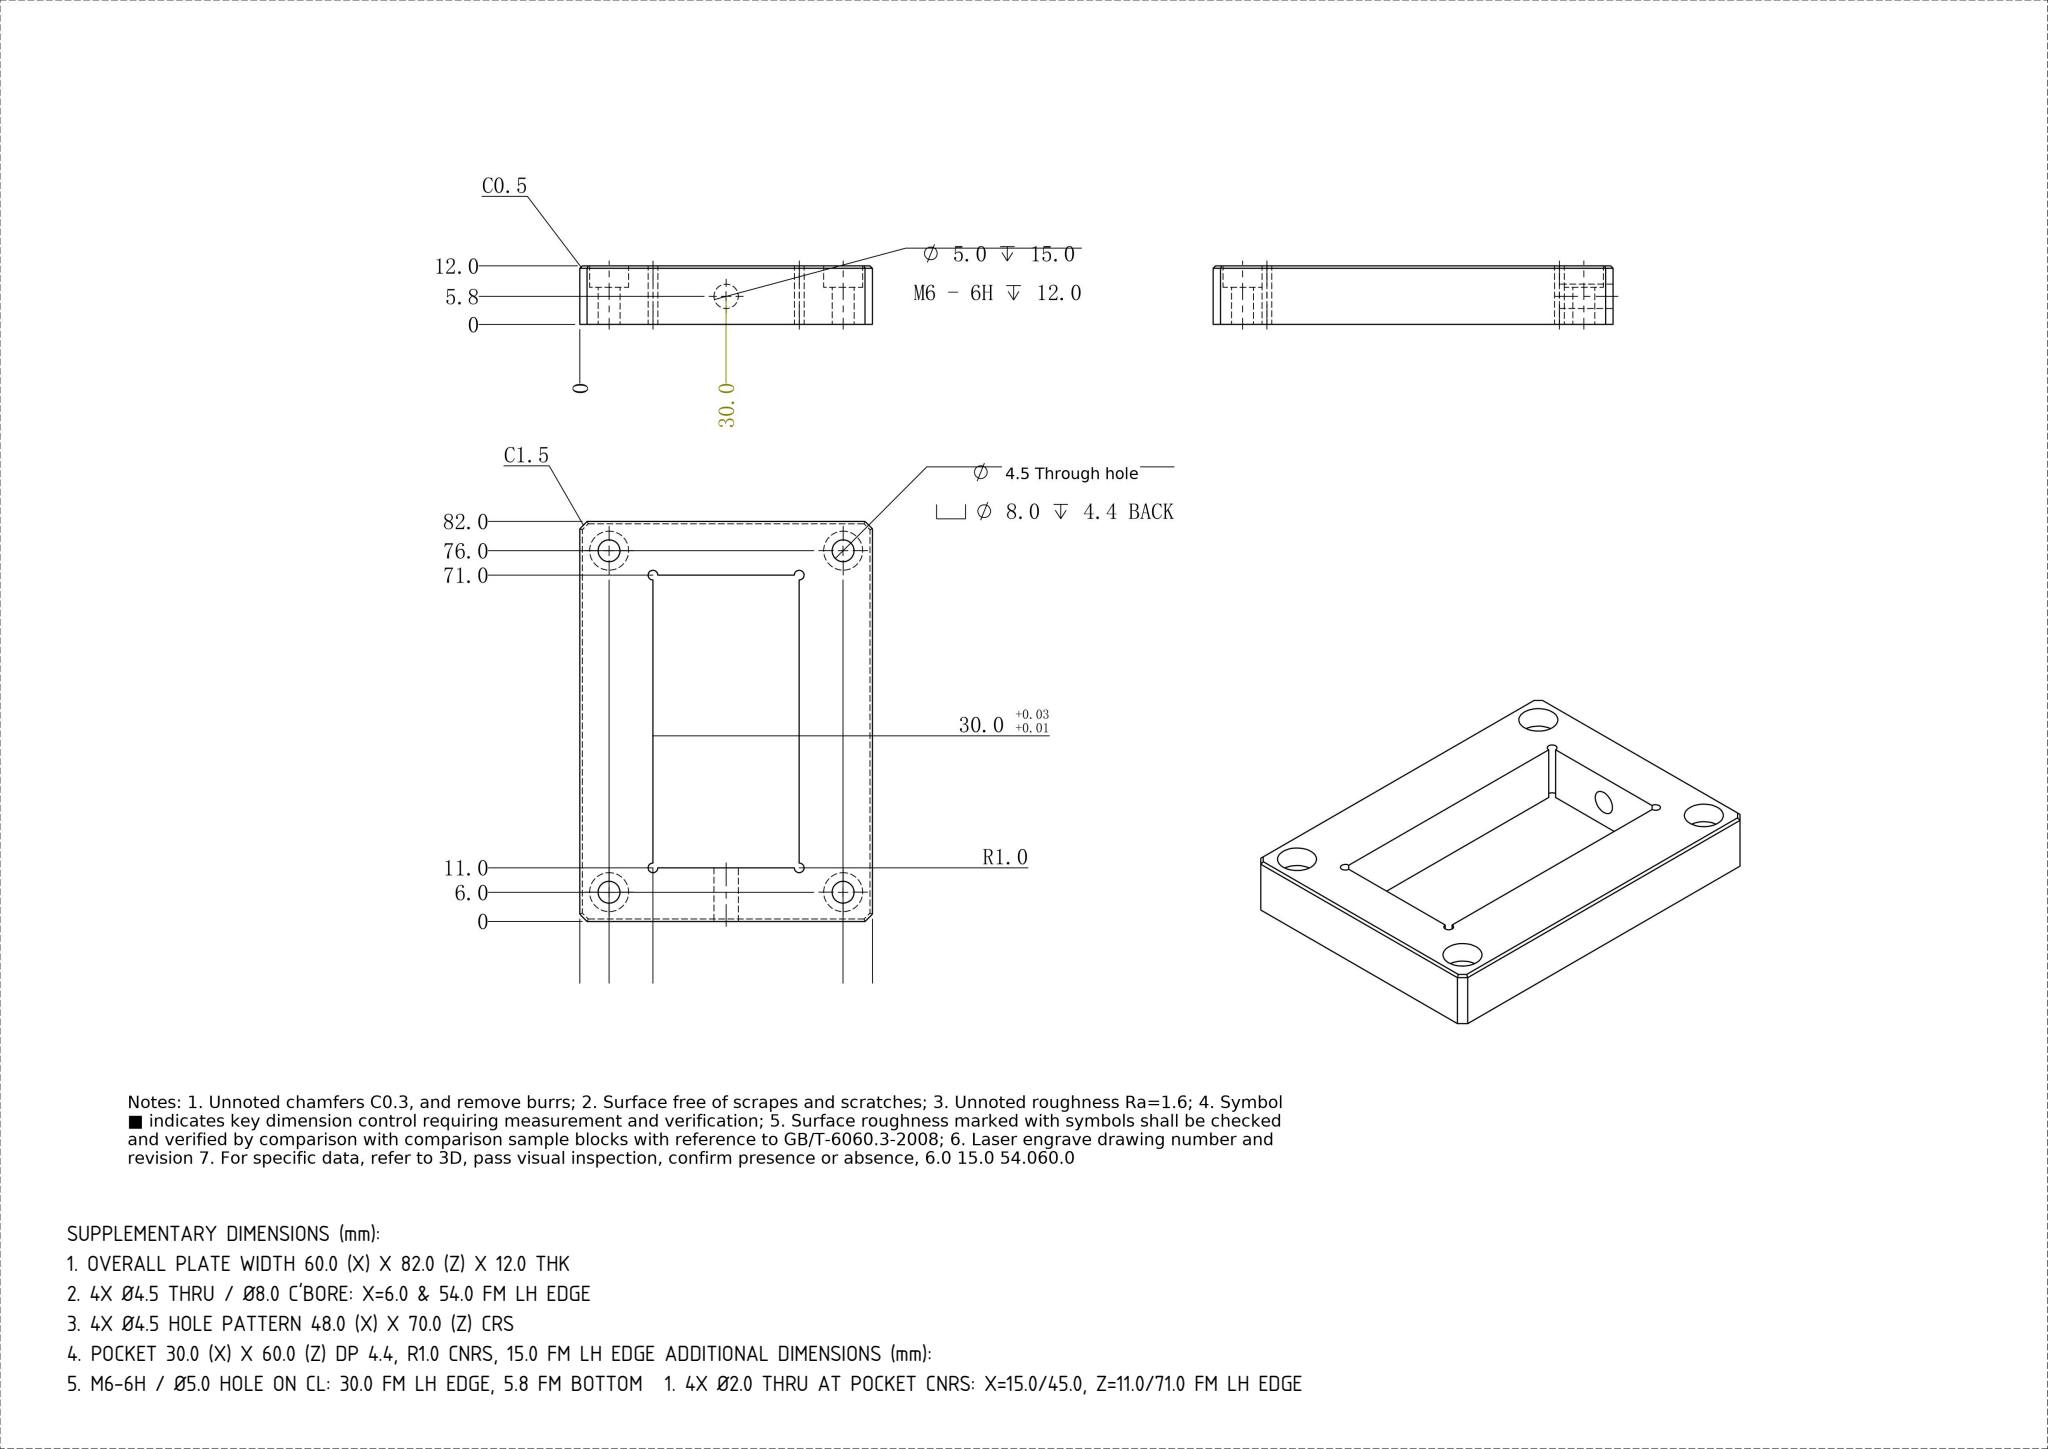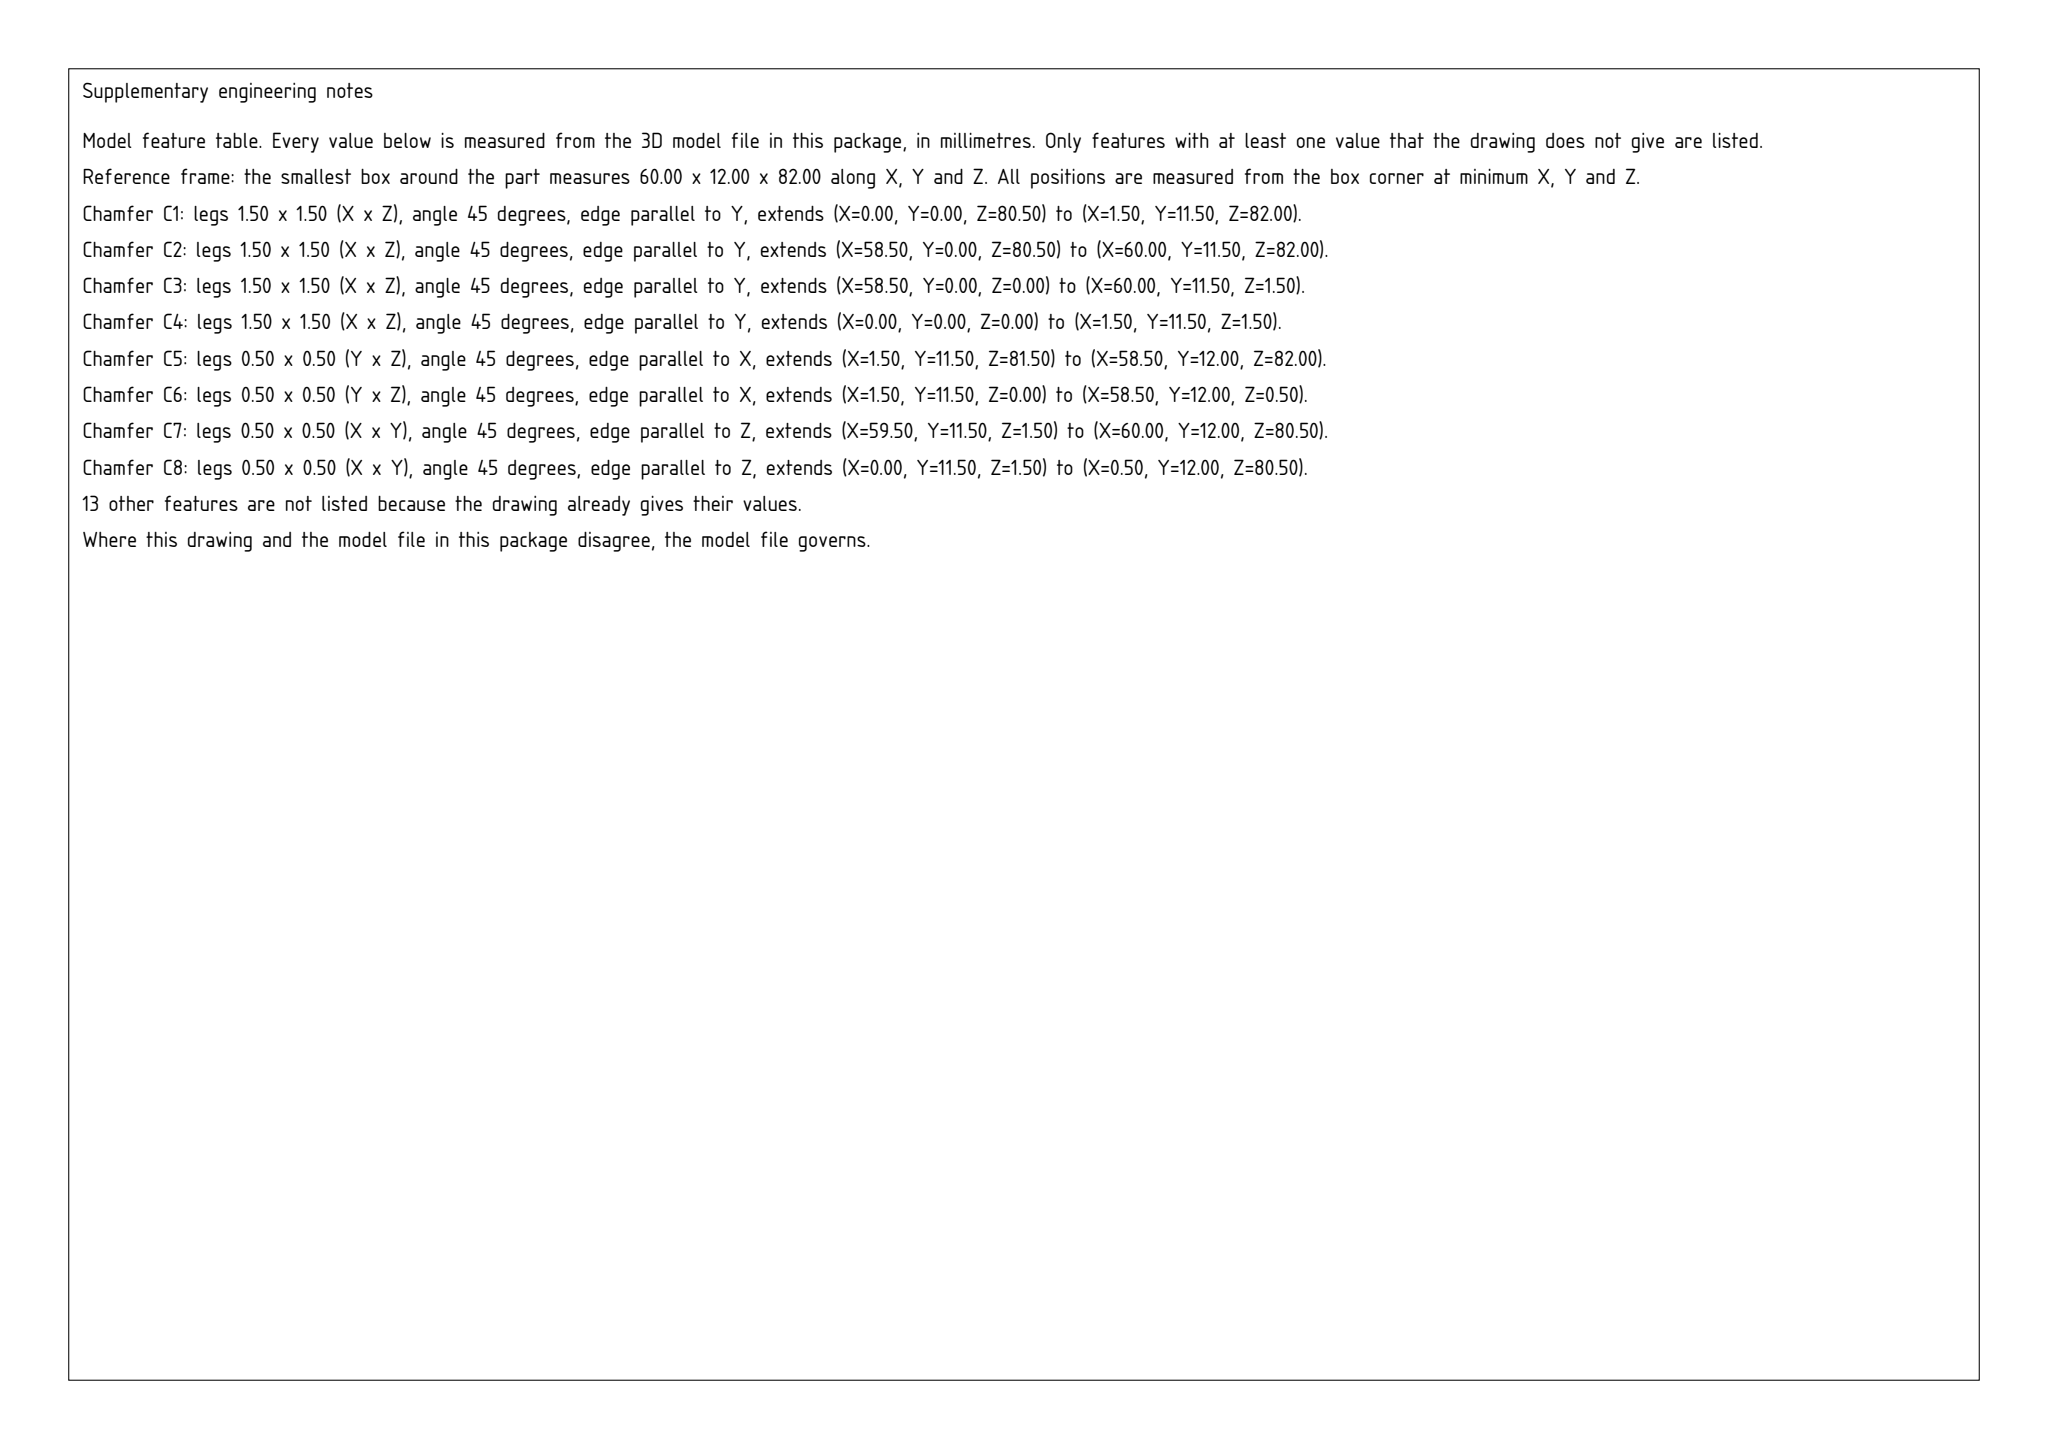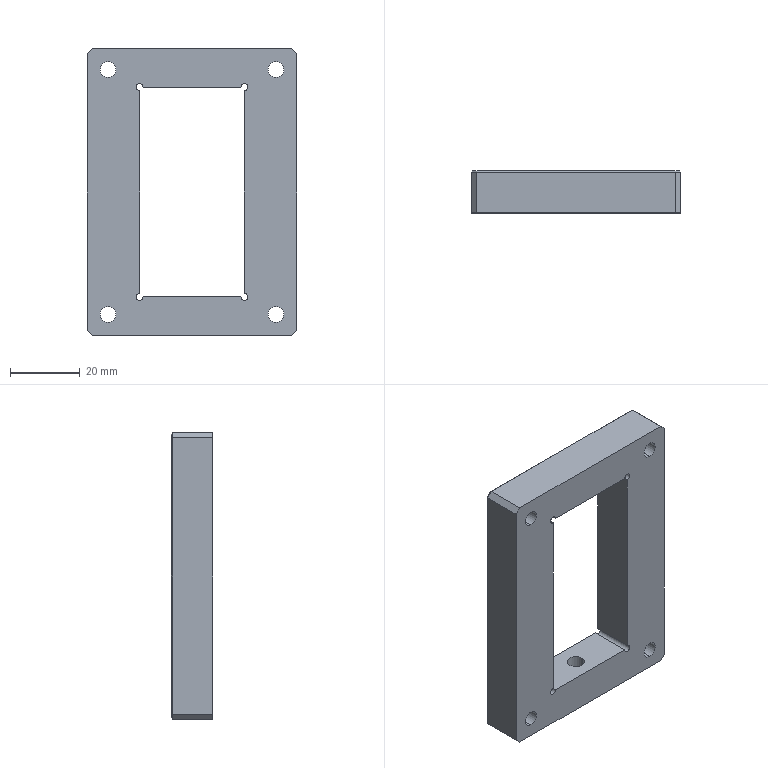Part | SolidWorks | mm | 1 solid | 50 faces | box 60 x 12 x 82 mm | volume 35654 mm3 | plane 26 | cylinder 24 | commonest cylinder face diameters 8 x8 4.5 x8 2 x6 5 x2
build123d program:
from build123d import *

# Parameters (mm, degrees)
SKETCH1_W                                       = 60
SKETCH1_H                                       = 12
BOSS_EXTRUDE1_DEPTH                             = 82
CHAMFER1_SIZE                                   = 1.5
CHAMFER2_SIZE                                   = 0.5
M4_HEX_SOCKET_HEAD_CAP_SCREW_CBORE1_D           = 4.5
M4_HEX_SOCKET_HEAD_CAP_SCREW_CBORE1_CBORE_D     = 8
M4_HEX_SOCKET_HEAD_CAP_SCREW_CBORE1_CBORE_DEPTH = 4.4
SKETCH6_W                                       = 30
SKETCH6_H                                       = 60
CUT_EXTRUDE1_DEPTH                              = 47
M6_TAPPED_HOLE1_D                               = 5
M6_TAPPED_HOLE1_DEPTH                           = 15
M6_TAPPED_HOLE1_TIP                             = 1.502
SKETCH9_R                                       = 1
CUT_EXTRUDE2_DEPTH                              = 47


with BuildPart() as part:
    # Sketch1 → Boss-Extrude1 (new body)
    with BuildSketch(Plane(origin=(0, 0, -5), x_dir=(-1, 0, 0), z_dir=(0, 0, -1))):
        with Locations((5, 0)):
            Rectangle(SKETCH1_W, SKETCH1_H)
    extrude(amount=-BOSS_EXTRUDE1_DEPTH)

    # Chamfer1
    chamfer1_edges = [part.edges().sort_by_distance(p)[0] for p in [
        (25, 0, 77),
        (-35, 0, 77),
        (25, 0, -5),
        (-35, 0, -5),
    ]]
    chamfer(chamfer1_edges, length=CHAMFER1_SIZE)

    # Chamfer2
    chamfer2_edges = [part.edges().sort_by_distance(p)[0] for p in [
        (-35, 6, 36),
        (-5, 6, -5),
        (-5, 6, 77),
        (25, 6, 36),
        (-34.25, 6, -4.25),
        (24.25, 6, -4.25),
        (24.25, 6, 76.25),
        (-34.25, 6, 76.25),
    ]]
    chamfer(chamfer2_edges, length=CHAMFER2_SIZE)

    # M4 Hex Socket Head Cap Screw CBORE1 (through all)
    with Locations(Plane(origin=(0, 6, 0), x_dir=(1, 0, 0), z_dir=(0, 1, 0))):
        with Locations((-29, -1), (19, -1), (-29, -71), (19, -71)):
            CounterBoreHole(M4_HEX_SOCKET_HEAD_CAP_SCREW_CBORE1_D / 2, M4_HEX_SOCKET_HEAD_CAP_SCREW_CBORE1_CBORE_D / 2, M4_HEX_SOCKET_HEAD_CAP_SCREW_CBORE1_CBORE_DEPTH)

    # Sketch6 → Cut-Extrude1 (cut)
    with BuildSketch(Plane(origin=(0, 6, 0), x_dir=(1, 0, 0), z_dir=(0, 1, 0))):
        with Locations((-5, -36)):
            Rectangle(SKETCH6_W, SKETCH6_H)
    extrude(amount=-CUT_EXTRUDE1_DEPTH, mode=Mode.SUBTRACT)

    # M6 Tapped Hole1
    with Locations(Plane(origin=(0, 0, -5), x_dir=(-1, 0, 0), z_dir=(0, 0, -1))):
        with Locations((5, -0.25)):
            Hole(M6_TAPPED_HOLE1_D / 2, depth=M6_TAPPED_HOLE1_DEPTH)
            with Locations((0, 0, -(M6_TAPPED_HOLE1_DEPTH + M6_TAPPED_HOLE1_TIP / 2))):  # 118° drill point
                Cone(0, M6_TAPPED_HOLE1_D / 2, M6_TAPPED_HOLE1_TIP, mode=Mode.SUBTRACT)

    # Sketch9 → Cut-Extrude2 (cut)
    with BuildSketch(Plane(origin=(0, 6, 0), x_dir=(1, 0, 0), z_dir=(0, 1, 0))):
        with Locations((-20, -6)):
            Circle(SKETCH9_R)
        with Locations((10, -6)):
            Circle(SKETCH9_R)
        with Locations((-20, -66)):
            Circle(SKETCH9_R)
        with Locations((10, -66)):
            Circle(SKETCH9_R)
    extrude(amount=-CUT_EXTRUDE2_DEPTH, mode=Mode.SUBTRACT)


solid = part.part